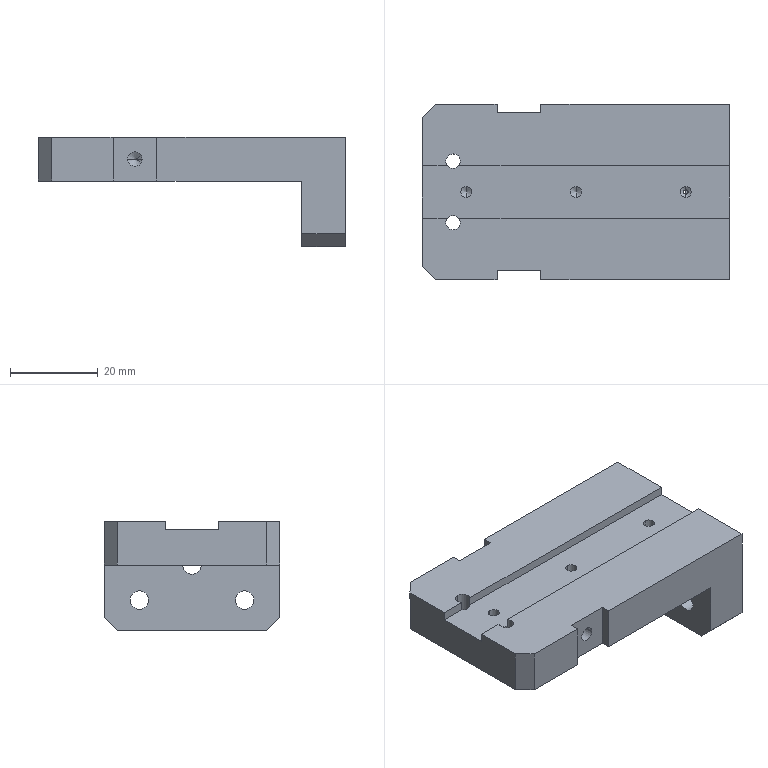Component | SolidWorks | 09HHHHHH2-1 | 1 solid | 57 faces | box 70 x 40 x 25 mm | volume 30893 mm3 | plane 26 | cylinder 20 | cone 11 | commonest cylinder face diameters 3.3 x8 4.2 x6 2.5 x6
build123d program:
from build123d import *

# Parameters (mm, degrees)
BOSS_EXTRUDE1_DEPTH   = 40
SKETCH2_W             = 12
SKETCH2_H             = 2
CUT_EXTRUDE1_DEPTH    = 91.677
M3_TAPPED_HOLE1_D     = 2.5
M3_TAPPED_HOLE1_DEPTH = 7.5
M3_TAPPED_HOLE1_TIP   = 0.7511
CHAMFER1_SIZE         = 3
M5_TAPPED_HOLE1_D     = 4.2
M5_TAPPED_HOLE1_DEPTH = 12.4
M5_TAPPED_HOLE1_TIP   = 1.262
M4_TAPPED_HOLE1_D     = 3.3
M4_TAPPED_HOLE1_DEPTH = 10.1
M4_TAPPED_HOLE1_TIP   = 0.9914
SKETCH9_W             = 10
SKETCH9_H             = 2
CUT_EXTRUDE2_DEPTH    = 635.116
M4_TAPPED_HOLE2_D     = 3.3
M4_TAPPED_HOLE2_DEPTH = 10.1
M4_TAPPED_HOLE2_TIP   = 0.9914
M4_TAPPED_HOLE3_D     = 3.3
M4_TAPPED_HOLE3_DEPTH = 10.1
M4_TAPPED_HOLE3_TIP   = 0.9914


with BuildPart() as part:
    # Sketch1 → Boss-Extrude1 (new body)
    with BuildSketch(Plane.XY):
        Polygon((562.359, -41.5), (562.359, -16.5), (632.359, -16.5), (632.359, -26.5), (572.359, -26.5), (572.359, -41.5), align=None)
    extrude(amount=-BOSS_EXTRUDE1_DEPTH)

    # Sketch2 → Cut-Extrude1 (cut, through all)
    with BuildSketch(Plane(origin=(632.359, 0, 0), x_dir=(0, 0, -1), z_dir=(1, 0, 0))):
        with Locations((20, -17.5)):
            Rectangle(SKETCH2_W, SKETCH2_H)
    extrude(amount=-CUT_EXTRUDE1_DEPTH, mode=Mode.SUBTRACT)

    # M3 Tapped Hole1
    with Locations(Plane(origin=(0, -16.5, 0), x_dir=(1, 0, 0), z_dir=(0, 1, 0))):
        with Locations((572.359, 20), (597.359, 20), (622.359, 20)):
            Hole(M3_TAPPED_HOLE1_D / 2, depth=M3_TAPPED_HOLE1_DEPTH)
            with Locations((0, 0, -(M3_TAPPED_HOLE1_DEPTH + M3_TAPPED_HOLE1_TIP / 2))):  # 118° drill point
                Cone(0, M3_TAPPED_HOLE1_D / 2, M3_TAPPED_HOLE1_TIP, mode=Mode.SUBTRACT)

    # Chamfer1
    chamfer1_edges = [part.edges().sort_by_distance(p)[0] for p in [
        (567.359, -41.5, -40),
        (632.359, -21.5, -40),
        (632.359, -21.5, 0),
        (567.359, -41.5, 0),
    ]]
    chamfer(chamfer1_edges, length=CHAMFER1_SIZE)

    # M5 Tapped Hole1
    with Locations(Plane.ZY.offset(-562.359)):
        with Locations((-32, -34.5), (-20, -26.5), (-8, -34.5)):
            Hole(M5_TAPPED_HOLE1_D / 2, depth=M5_TAPPED_HOLE1_DEPTH)
            with Locations((0, 0, -(M5_TAPPED_HOLE1_DEPTH + M5_TAPPED_HOLE1_TIP / 2))):  # 118° drill point
                Cone(0, M5_TAPPED_HOLE1_D / 2, M5_TAPPED_HOLE1_TIP, mode=Mode.SUBTRACT)

    # M4 Tapped Hole1
    with Locations(Plane(origin=(0, -26.5, 0), x_dir=(-1, 0, 0), z_dir=(0, -1, 0))):
        with Locations((-625.359, 13), (-625.359, 27)):
            Hole(M4_TAPPED_HOLE1_D / 2, depth=M4_TAPPED_HOLE1_DEPTH)
            with Locations((0, 0, -(M4_TAPPED_HOLE1_DEPTH + M4_TAPPED_HOLE1_TIP / 2))):  # 118° drill point
                Cone(0, M4_TAPPED_HOLE1_D / 2, M4_TAPPED_HOLE1_TIP, mode=Mode.SUBTRACT)

    # Sketch9 → Cut-Extrude2 (cut, through all)
    with BuildSketch(Plane(origin=(0, -16.5, 0), x_dir=(1, 0, 0), z_dir=(0, 1, 0))):
        with Locations((610.359, 1)):
            Rectangle(SKETCH9_W, SKETCH9_H)
        with Locations((610.359, 39)):
            Rectangle(SKETCH9_W, SKETCH9_H)
    extrude(amount=-CUT_EXTRUDE2_DEPTH, mode=Mode.SUBTRACT)

    # M4 Tapped Hole2
    with Locations(Plane.XY.offset(-2)):
        with Locations((610.359, -21.5)):
            Hole(M4_TAPPED_HOLE2_D / 2, depth=M4_TAPPED_HOLE2_DEPTH)
            with Locations((0, 0, -(M4_TAPPED_HOLE2_DEPTH + M4_TAPPED_HOLE2_TIP / 2))):  # 118° drill point
                Cone(0, M4_TAPPED_HOLE2_D / 2, M4_TAPPED_HOLE2_TIP, mode=Mode.SUBTRACT)

    # M4 Tapped Hole3
    with Locations(Plane(origin=(0, 0, -40), x_dir=(-1, 0, 0), z_dir=(0, 0, -1))):
        with Locations((-610.359, -21.5)):
            Hole(M4_TAPPED_HOLE3_D / 2, depth=M4_TAPPED_HOLE3_DEPTH)
            with Locations((0, 0, -(M4_TAPPED_HOLE3_DEPTH + M4_TAPPED_HOLE3_TIP / 2))):  # 118° drill point
                Cone(0, M4_TAPPED_HOLE3_D / 2, M4_TAPPED_HOLE3_TIP, mode=Mode.SUBTRACT)


solid = part.part

# Placed as in the assembly
solid = solid.moved(Location((-8, -266.383, 6.344), (-90, 0, 180)))